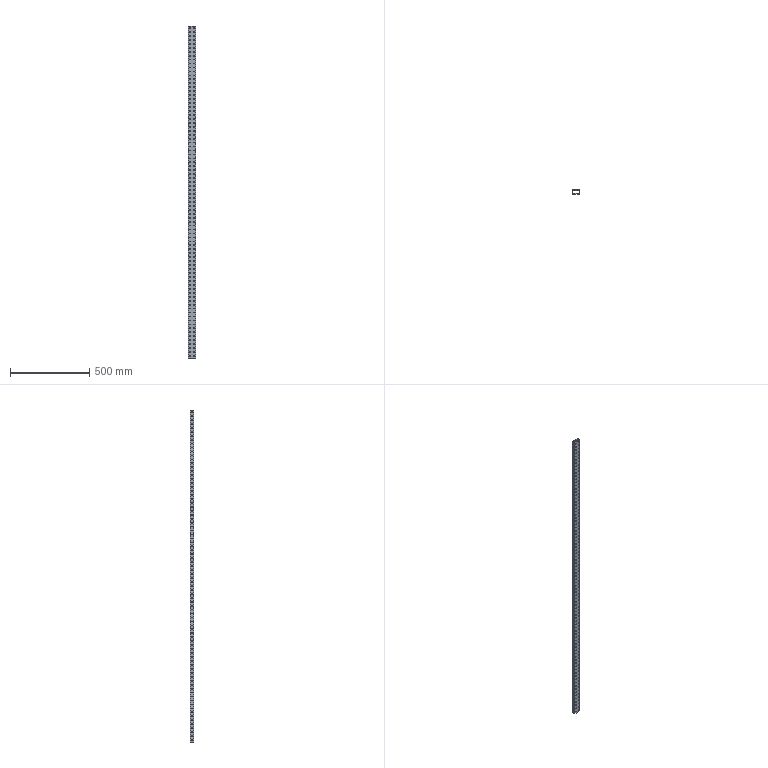Component | SolidWorks | MiddleColumn-2 | 1 solid | 1046 faces | volume 509687 mm3 | cylinder 1016 | plane 30 | commonest cylinder face diameters 5 x1008 6 x4 2 x4 | material Plain Carbon Steel